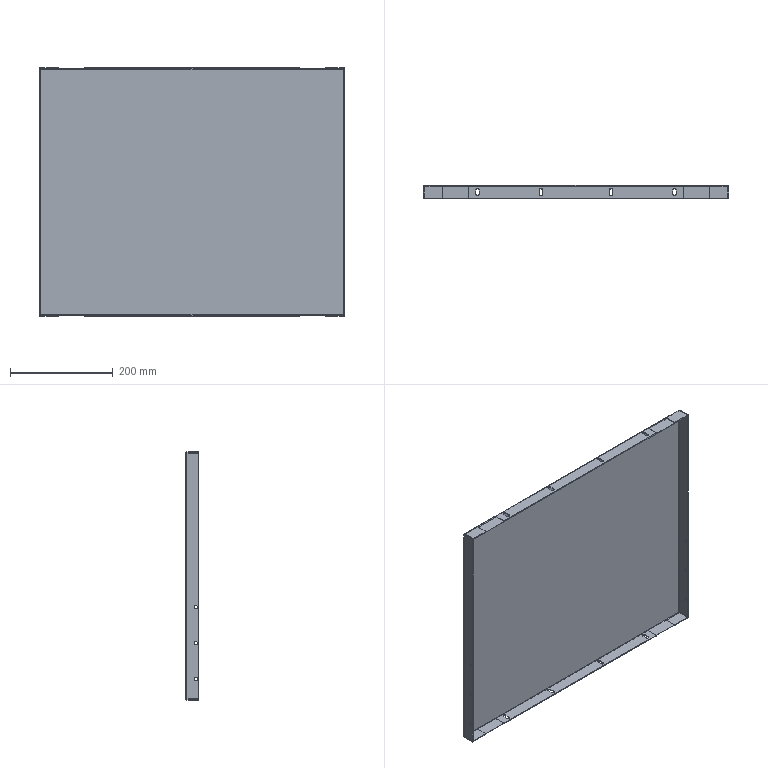Component | SolidWorks | 01-10ElectricalControlPanel-1 | 1 solid | 142 faces | volume 661656 mm3 | plane 66 | cylinder 56 | spline 20 | commonest cylinder face diameters 6.5 x24 6 x12 4 x8 5.473 x4 1.473 x4 2 x4 | material SGLCC